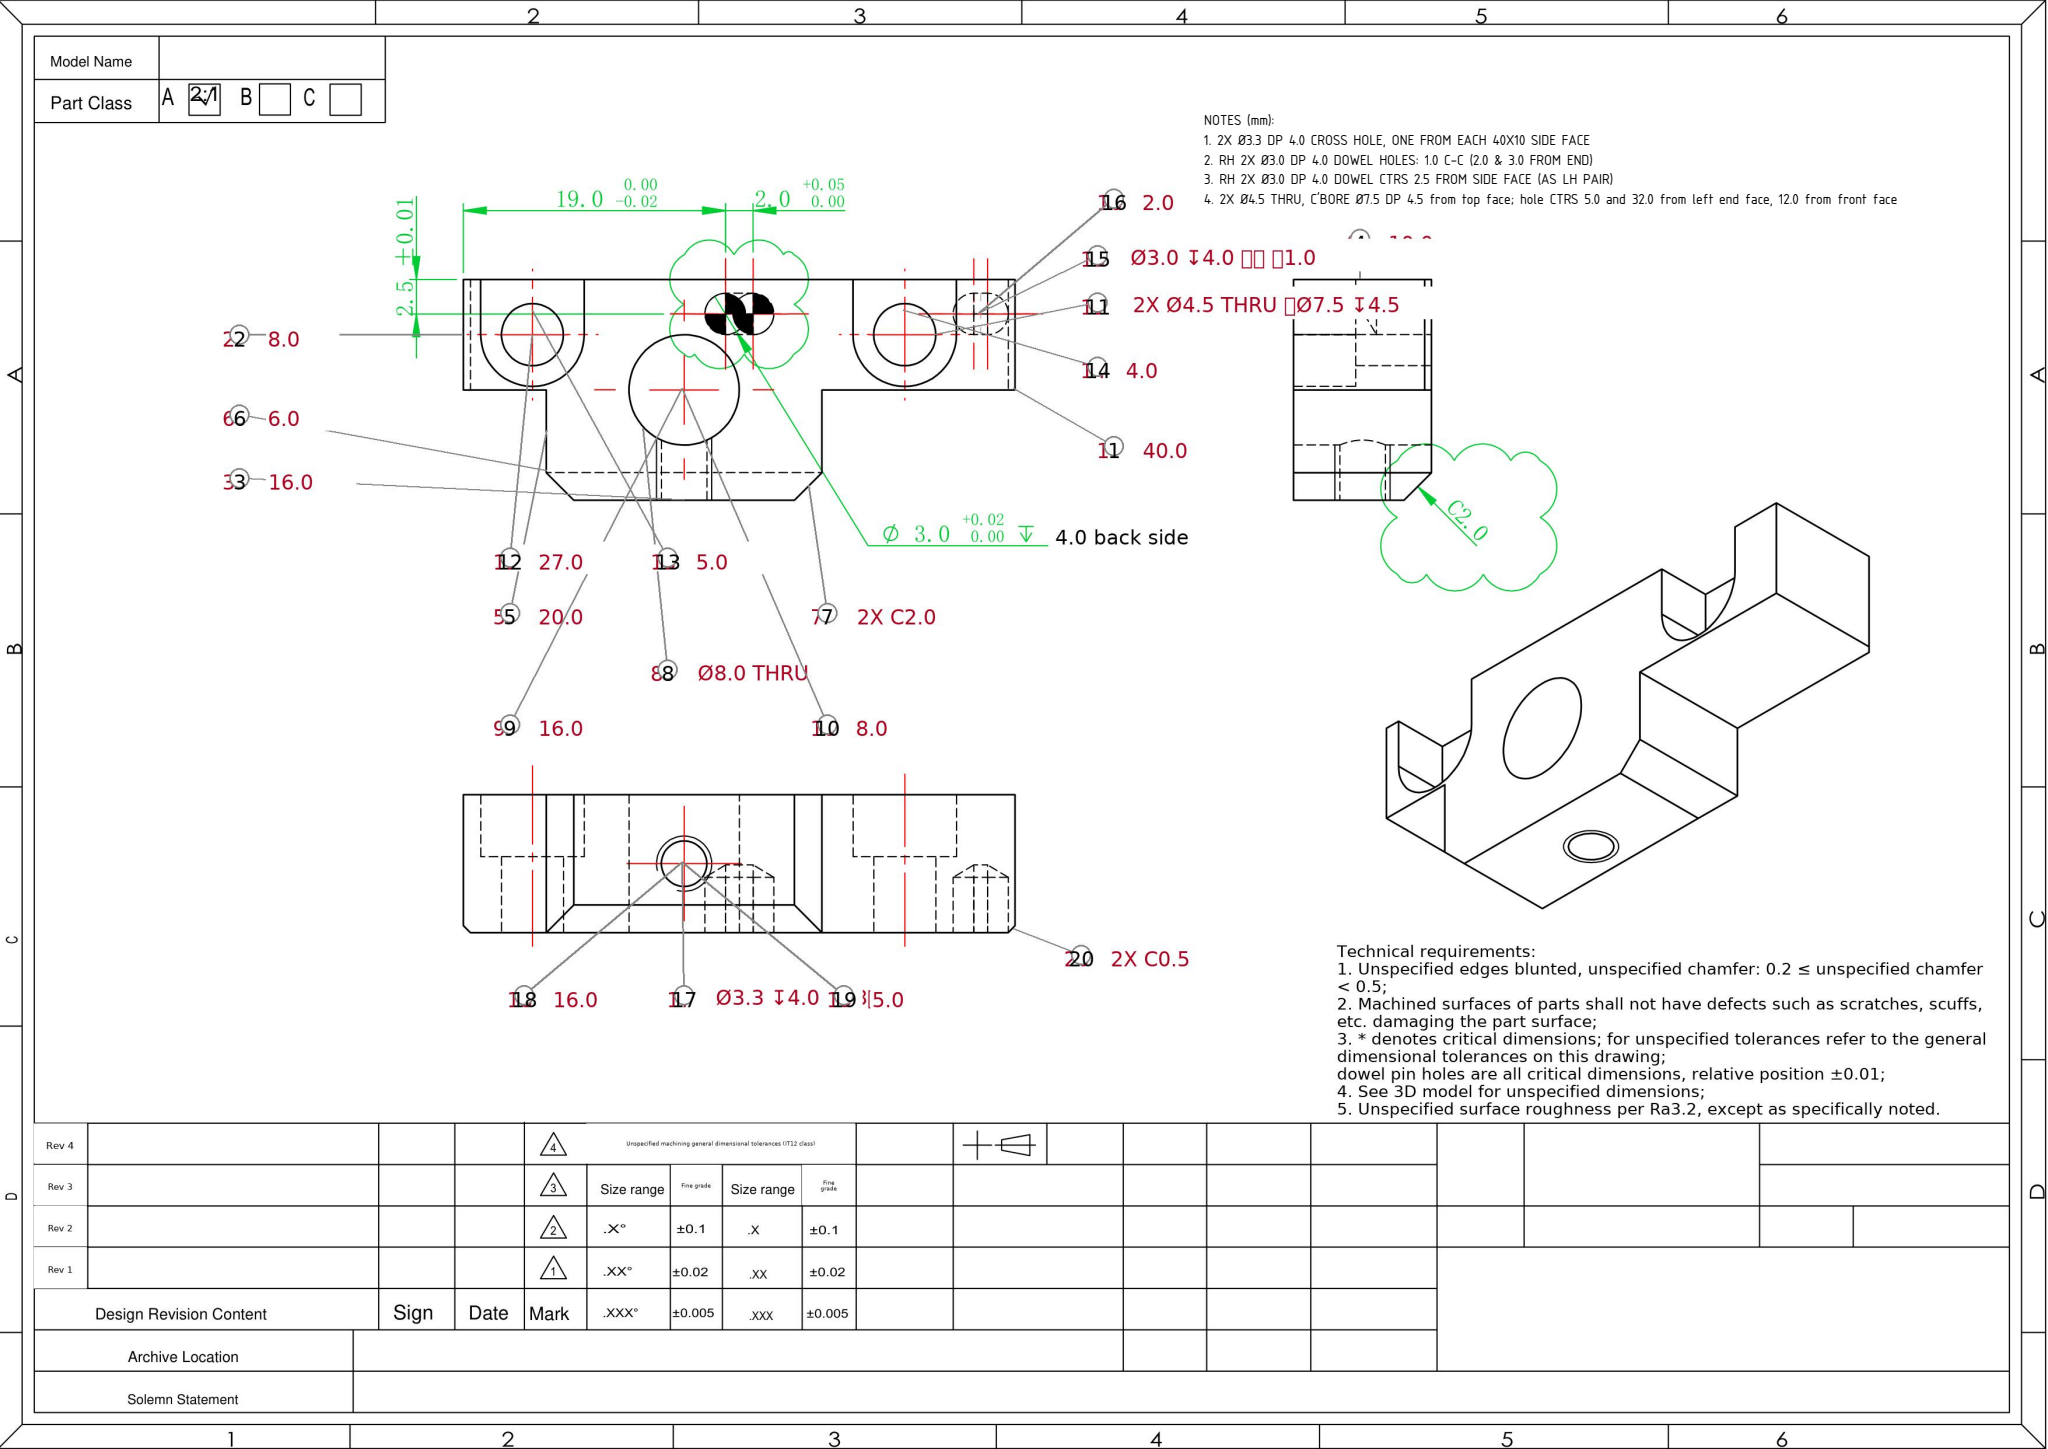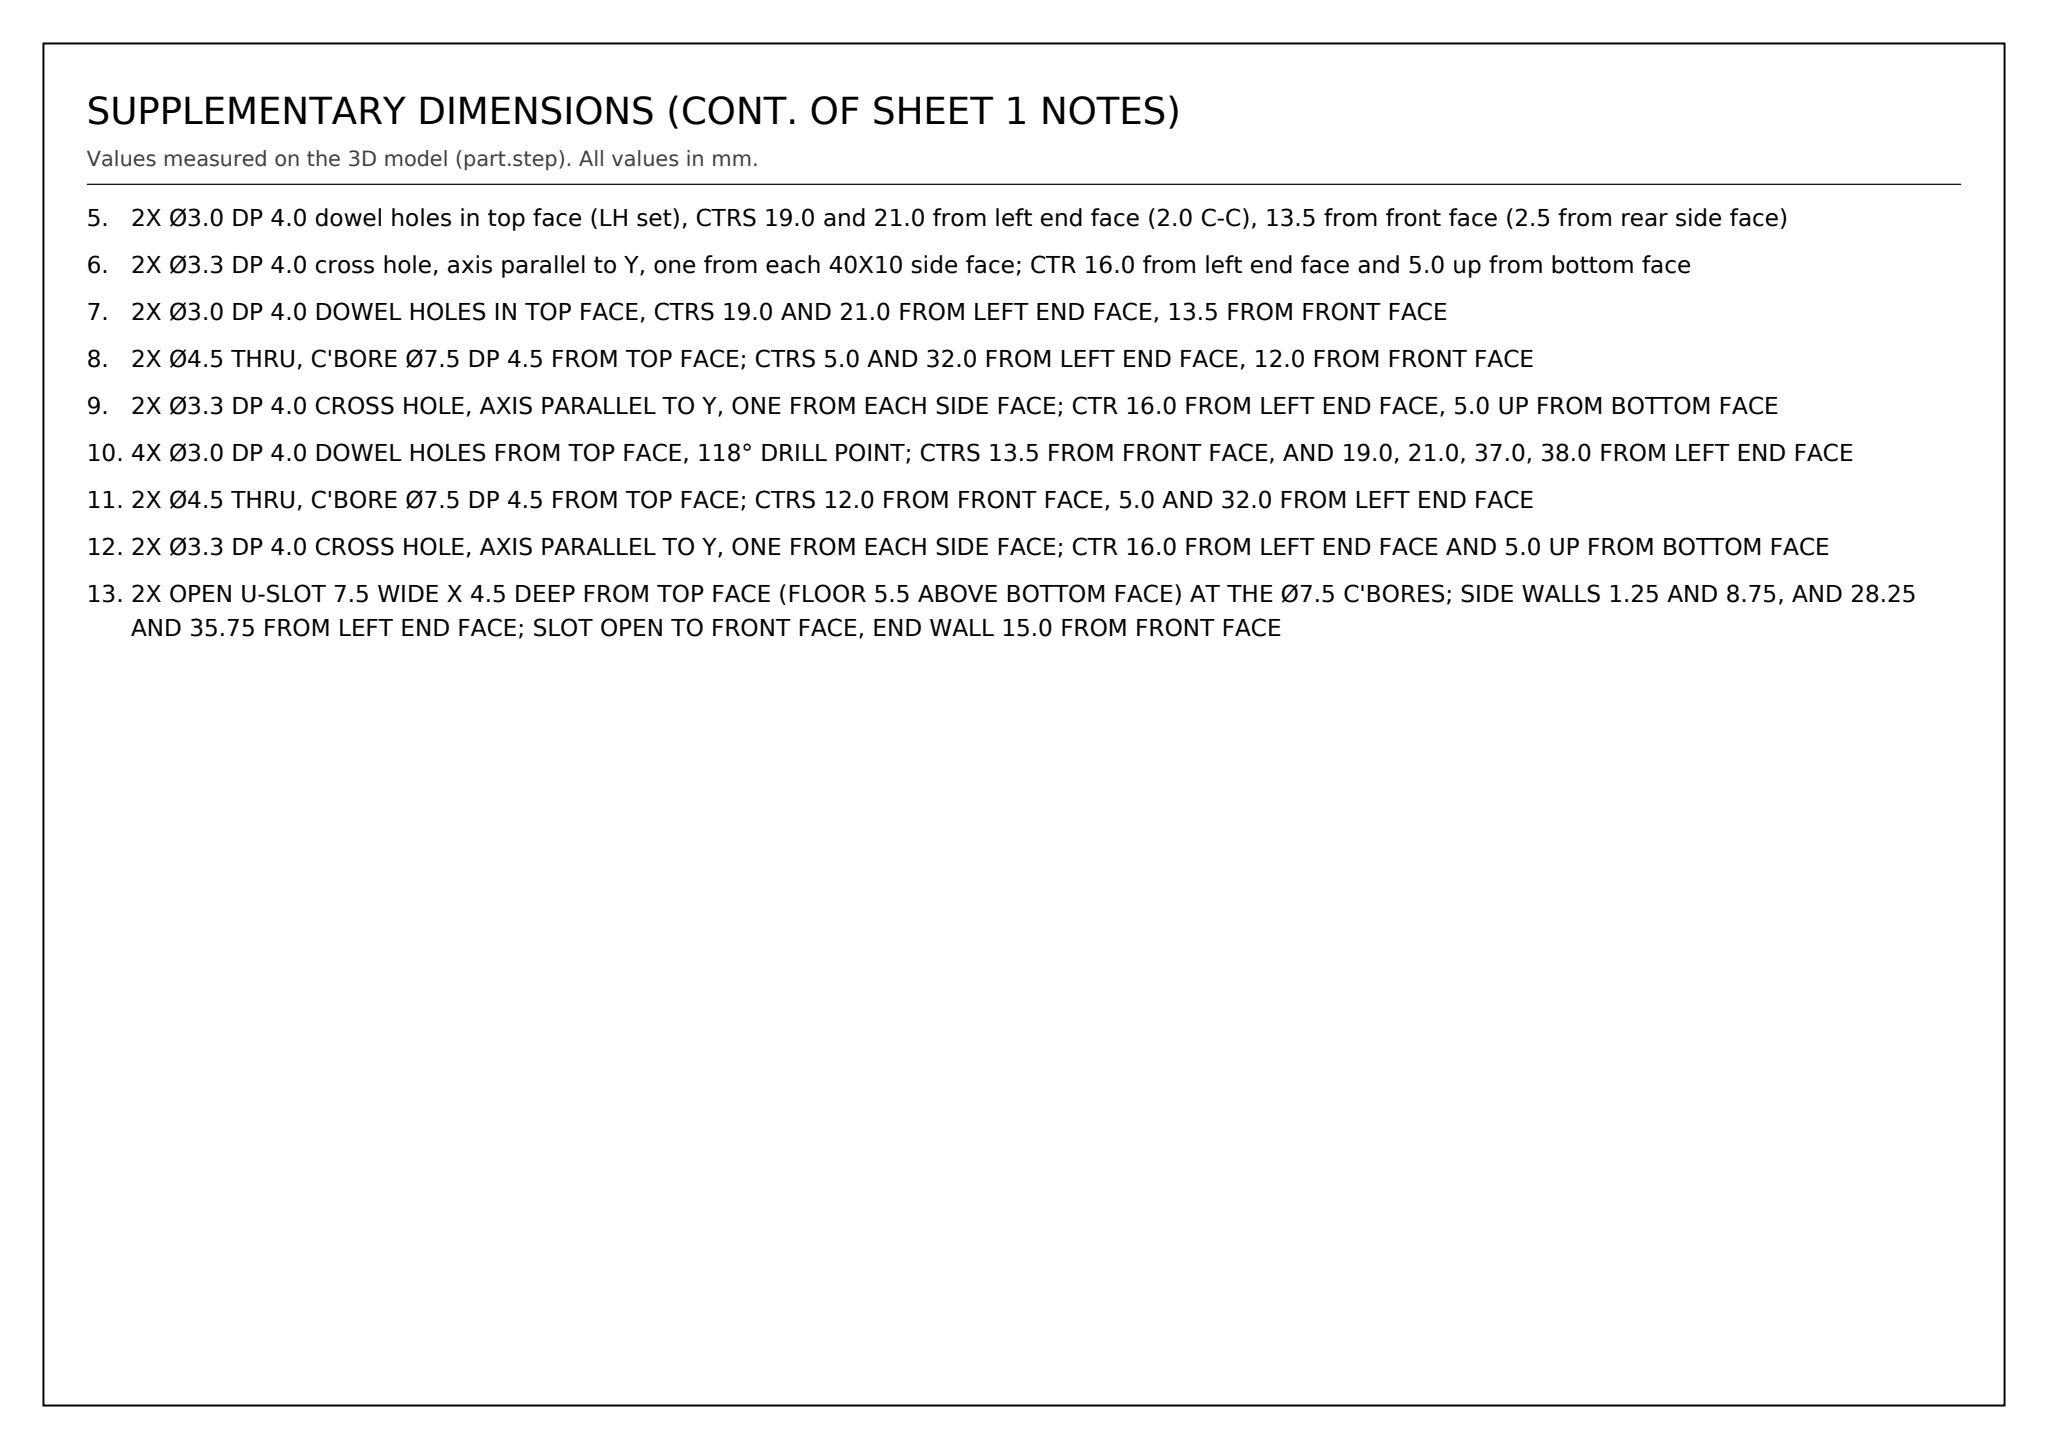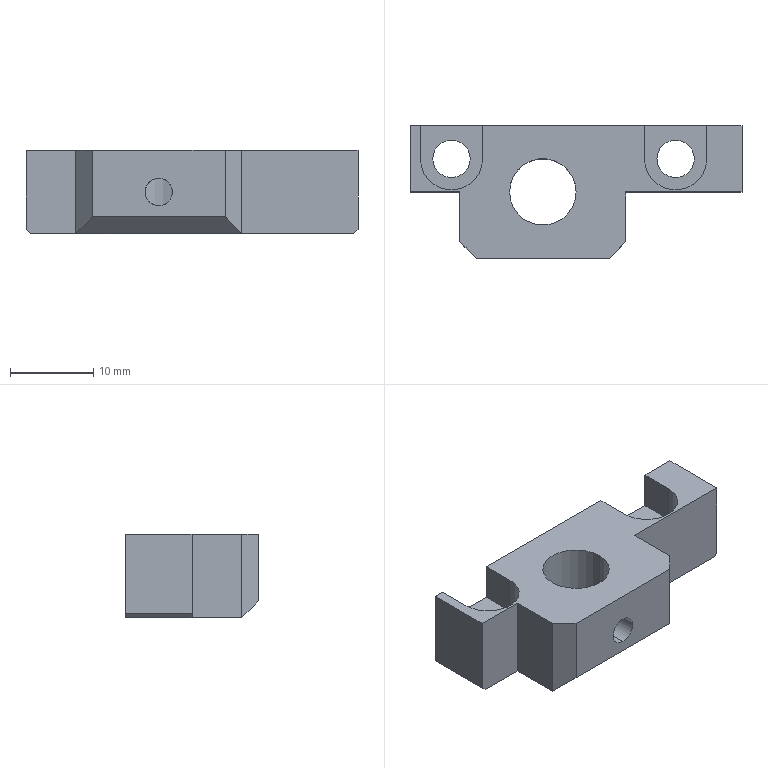Part | SolidWorks | mm | 1 solid | 51 faces | box 40 x 16 x 10 mm | volume 3441 mm3 | plane 29 | cylinder 16 | cone 6 | commonest cylinder face diameters 3 x6 4.5 x4 3.3 x2 8 x2 7.5 x2
Drawing notes:
2X Ø3.3 DP 4.0 CROSS HOLE, ONE FROM EACH 40X10 SIDE FACE | from the solid: cyl dia 3.3 axis y at x=16.0, z=5.0, len 4.36, count 2; y-faces at y=0 and y=16 (bbox 40x16x10)
RH 2X Ø3.0 DP 4.0 DOWEL HOLES: 1.0 C-C (2.0 & 3.0 FROM END) | from the solid: cyl dia 3.0 axis z at x=37.0 and x=38.0, y=13.5, depth 4.0; bbox x=40 end face
RH 2X Ø3.0 DP 4.0 DOWEL CTRS 2.5 FROM SIDE FACE (AS LH PAIR) | from the solid: cyl dia 3.0 axis z at y=13.5; side face plane y=16.0 -> 16.0-13.5=2.5
2X Ø4.5 THRU, C'BORE Ø7.5 DP 4.5 from top face; hole CTRS 5.0 and 32.0 from left end face, 12.0 from front face | from the solid: cylinders dia 4.5 axis z at (5.0,12.0) and (32.0,12.0) len 5.5; cylinders dia 7.5 axis z at (5.0,12.0) and (32.0,12.0) len 4.5
2X Ø3.0 DP 4.0 dowel holes in top face (LH set), CTRS 19.0 and 21.0 from left end face (2.0 C-C), 13.5 from front face (2.5 from rear side face) | from the solid: cylinders dia 3.0 axis z at (19.0,13.5) and (21.0,13.5), length 4.0
2X Ø3.3 DP 4.0 cross hole, axis parallel to Y, one from each 40X10 side face; CTR 16.0 from left end face and 5.0 up from bottom face | from the solid: cylinders dia 3.3 axis y at (16.0, z=5.0), length 4.36; cones 118° ref dia 3.0 (drill point)
2X Ø3.0 DP 4.0 DOWEL HOLES IN TOP FACE, CTRS 19.0 AND 21.0 FROM LEFT END FACE, 13.5 FROM FRONT FACE | from the solid: cylinders dia 3.0 axis z at (19.0,13.5) and (21.0,13.5), length 4.0; bbox 40x16x10
2X Ø4.5 THRU, C'BORE Ø7.5 DP 4.5 FROM TOP FACE; CTRS 5.0 AND 32.0 FROM LEFT END FACE, 12.0 FROM FRONT FACE | from the solid: cylinders dia 4.5 axis z at (5.0,12.0) and (32.0,12.0) length 5.5; dia 7.5 axis z at same positions length 4.5
2X Ø3.3 DP 4.0 CROSS HOLE, AXIS PARALLEL TO Y, ONE FROM EACH SIDE FACE; CTR 16.0 FROM LEFT END FACE, 5.0 UP FROM BOTTOM FACE | from the solid: cylinders dia 3.3 axis y at (x=16.0, z=5.0), length 4.36, count 2
4X Ø3.0 DP 4.0 DOWEL HOLES FROM TOP FACE, 118° DRILL POINT; CTRS 13.5 FROM FRONT FACE, AND 19.0, 21.0, 37.0, 38.0 FROM LEFT END FACE | from the solid: cylinders dia 3.0 axis z at (19.0,13.5),(21.0,13.5),(37.0,13.5),(38.0,13.5), length 4.0; cones 118° ref dia 3.0
2X Ø4.5 THRU, C'BORE Ø7.5 DP 4.5 FROM TOP FACE; CTRS 12.0 FROM FRONT FACE, 5.0 AND 32.0 FROM LEFT END FACE | from the solid: cylinders dia 4.5 axis z at (5.0,12.0) and (32.0,12.0) length 5.5; dia 7.5 axis z at same positions length 4.5
2X Ø3.3 DP 4.0 CROSS HOLE, AXIS PARALLEL TO Y, ONE FROM EACH SIDE FACE; CTR 16.0 FROM LEFT END FACE AND 5.0 UP FROM BOTTOM FACE | from the solid: cylinders dia 3.3 axis y at (16.0, z=5.0), length 4.36, count 2
2X OPEN U-SLOT 7.5 WIDE X 4.5 DEEP FROM TOP FACE (FLOOR 5.5 ABOVE BOTTOM FACE) AT THE Ø7.5 C'BORES; SIDE WALLS 1.25 AND 8.75, AND 28.25 AND 35.75 FROM LEFT END FACE; SLOT OPEN TO FRONT FACE, END WALL 15.0 FROM FRONT FACE | from the solid: axis planes x=1.25, 8.75, 28.25, 35.75; y=15.0 (2); z=5.5 (2); bbox 40.0x16.0x10.0